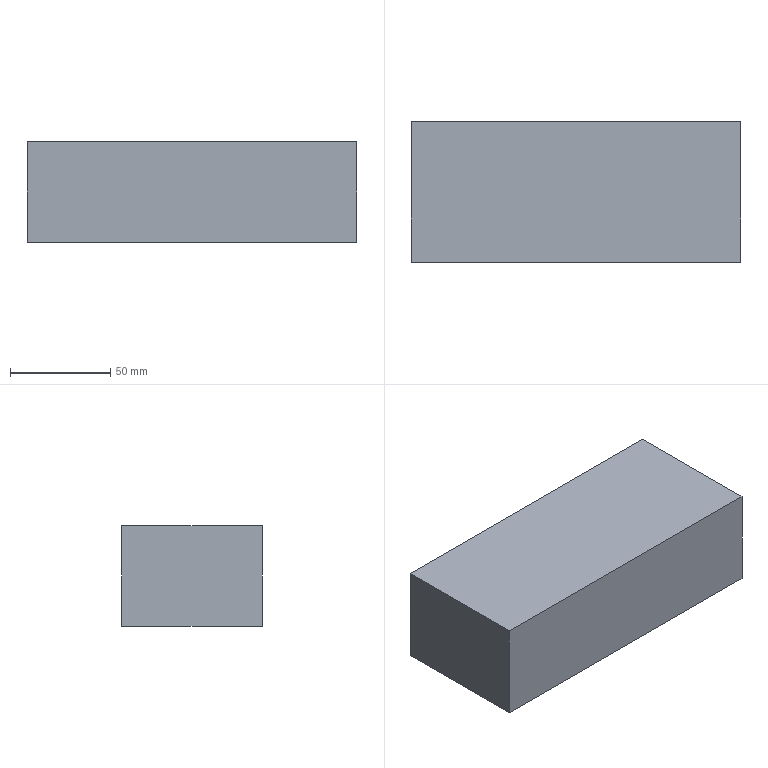Component | NX | PEN_HOLDER_BLOCK | 1 solid | 6 faces | box 164 x 70 x 50 mm | volume 574000 mm3 | plane 6
STEP:
#1=CARTESIAN_POINT('',(0.,0.,0.));
#2=DIRECTION('',(0.,0.,1.));
#3=DIRECTION('',(1.,0.,0.));
#4=AXIS2_PLACEMENT_3D('',#1,#2,#3);
#5=CARTESIAN_POINT('',(289.534,43.893,-32.704));
#6=VERTEX_POINT('',#5);
#7=CARTESIAN_POINT('',(289.534,43.893,17.296));
#8=VERTEX_POINT('',#7);
#9=CARTESIAN_POINT('',(289.534,43.893,-32.704));
#10=DIRECTION('',(0.,0.,1.));
#11=VECTOR('',#10,1.);
#12=LINE('',#9,#11);
#13=CARTESIAN_POINT('',(125.534,43.893,-32.704));
#14=DIRECTION('',(0.,1.,0.));
#15=DIRECTION('',(1.,0.,0.));
#16=AXIS2_PLACEMENT_3D('',#13,#14,#15);
#17=PLANE('',#16);
#18=CARTESIAN_POINT('',(164.,0.));
#19=DIRECTION('',(0.,-1.));
#20=VECTOR('',#19,1.);
#21=LINE('',#18,#20);
#22=(GEOMETRIC_REPRESENTATION_CONTEXT(2)PARAMETRIC_REPRESENTATION_CONTEXT()REPRESENTATION_CONTEXT('',''));
#23=DEFINITIONAL_REPRESENTATION('',(#21),#22);
#24=PCURVE('',#17,#23);
#25=CARTESIAN_POINT('',(289.534,103.893,-7.704));
#26=DIRECTION('',(-1.,0.,0.));
#27=DIRECTION('',(0.,1.,0.));
#28=AXIS2_PLACEMENT_3D('',#25,#26,#27);
#29=PLANE('',#28);
#30=CARTESIAN_POINT('',(-60.,25.));
#31=DIRECTION('',(0.,-1.));
#32=VECTOR('',#31,1.);
#33=LINE('',#30,#32);
#34=(GEOMETRIC_REPRESENTATION_CONTEXT(2)PARAMETRIC_REPRESENTATION_CONTEXT()REPRESENTATION_CONTEXT('',''));
#35=DEFINITIONAL_REPRESENTATION('',(#33),#34);
#36=PCURVE('',#29,#35);
#37=SURFACE_CURVE('',#12,(#24,#36),.PCURVE_S1.);
#38=EDGE_CURVE('',#6,#8,#37,.T.);
#39=ORIENTED_EDGE('',*,*,#38,.T.);
#40=CARTESIAN_POINT('',(125.534,43.893,17.296));
#41=VERTEX_POINT('',#40);
#42=CARTESIAN_POINT('',(125.534,43.893,17.296));
#43=DIRECTION('',(1.,0.,0.));
#44=VECTOR('',#43,1.);
#45=LINE('',#42,#44);
#46=CARTESIAN_POINT('',(0.,-50.));
#47=DIRECTION('',(1.,0.));
#48=VECTOR('',#47,1.);
#49=LINE('',#46,#48);
#50=(GEOMETRIC_REPRESENTATION_CONTEXT(2)PARAMETRIC_REPRESENTATION_CONTEXT()REPRESENTATION_CONTEXT('',''));
#51=DEFINITIONAL_REPRESENTATION('',(#49),#50);
#52=PCURVE('',#17,#51);
#53=CARTESIAN_POINT('',(125.534,43.893,17.296));
#54=DIRECTION('',(0.,0.,-1.));
#55=DIRECTION('',(-1.,0.,0.));
#56=AXIS2_PLACEMENT_3D('',#53,#54,#55);
#57=PLANE('',#56);
#58=CARTESIAN_POINT('',(0.,0.));
#59=DIRECTION('',(-1.,0.));
#60=VECTOR('',#59,1.);
#61=LINE('',#58,#60);
#62=(GEOMETRIC_REPRESENTATION_CONTEXT(2)PARAMETRIC_REPRESENTATION_CONTEXT()REPRESENTATION_CONTEXT('',''));
#63=DEFINITIONAL_REPRESENTATION('',(#61),#62);
#64=PCURVE('',#57,#63);
#65=SURFACE_CURVE('',#45,(#52,#64),.PCURVE_S1.);
#66=EDGE_CURVE('',#41,#8,#65,.T.);
#67=ORIENTED_EDGE('',*,*,#66,.F.);
#68=CARTESIAN_POINT('',(125.534,43.893,-32.704));
#69=VERTEX_POINT('',#68);
#70=CARTESIAN_POINT('',(125.534,43.893,-32.704));
#71=DIRECTION('',(0.,0.,1.));
#72=VECTOR('',#71,1.);
#73=LINE('',#70,#72);
#74=CARTESIAN_POINT('',(0.,0.));
#75=DIRECTION('',(0.,-1.));
#76=VECTOR('',#75,1.);
#77=LINE('',#74,#76);
#78=(GEOMETRIC_REPRESENTATION_CONTEXT(2)PARAMETRIC_REPRESENTATION_CONTEXT()REPRESENTATION_CONTEXT('',''));
#79=DEFINITIONAL_REPRESENTATION('',(#77),#78);
#80=PCURVE('',#17,#79);
#81=CARTESIAN_POINT('',(125.534,103.893,-7.704));
#82=DIRECTION('',(-1.,0.,0.));
#83=DIRECTION('',(0.,1.,0.));
#84=AXIS2_PLACEMENT_3D('',#81,#82,#83);
#85=PLANE('',#84);
#86=CARTESIAN_POINT('',(-60.,25.));
#87=DIRECTION('',(0.,-1.));
#88=VECTOR('',#87,1.);
#89=LINE('',#86,#88);
#90=(GEOMETRIC_REPRESENTATION_CONTEXT(2)PARAMETRIC_REPRESENTATION_CONTEXT()REPRESENTATION_CONTEXT('',''));
#91=DEFINITIONAL_REPRESENTATION('',(#89),#90);
#92=PCURVE('',#85,#91);
#93=SURFACE_CURVE('',#73,(#80,#92),.PCURVE_S1.);
#94=EDGE_CURVE('',#69,#41,#93,.T.);
#95=ORIENTED_EDGE('',*,*,#94,.F.);
#96=CARTESIAN_POINT('',(125.534,43.893,-32.704));
#97=DIRECTION('',(1.,0.,0.));
#98=VECTOR('',#97,1.);
#99=LINE('',#96,#98);
#100=CARTESIAN_POINT('',(0.,0.));
#101=DIRECTION('',(1.,0.));
#102=VECTOR('',#101,1.);
#103=LINE('',#100,#102);
#104=(GEOMETRIC_REPRESENTATION_CONTEXT(2)PARAMETRIC_REPRESENTATION_CONTEXT()REPRESENTATION_CONTEXT('',''));
#105=DEFINITIONAL_REPRESENTATION('',(#103),#104);
#106=PCURVE('',#17,#105);
#107=CARTESIAN_POINT('',(125.534,163.893,-32.704));
#108=DIRECTION('',(0.,0.,1.));
#109=DIRECTION('',(1.,0.,0.));
#110=AXIS2_PLACEMENT_3D('',#107,#108,#109);
#111=PLANE('',#110);
#112=CARTESIAN_POINT('',(0.,-120.));
#113=DIRECTION('',(1.,0.));
#114=VECTOR('',#113,1.);
#115=LINE('',#112,#114);
#116=(GEOMETRIC_REPRESENTATION_CONTEXT(2)PARAMETRIC_REPRESENTATION_CONTEXT()REPRESENTATION_CONTEXT('',''));
#117=DEFINITIONAL_REPRESENTATION('',(#115),#116);
#118=PCURVE('',#111,#117);
#119=SURFACE_CURVE('',#99,(#106,#118),.PCURVE_S1.);
#120=EDGE_CURVE('',#69,#6,#119,.T.);
#121=ORIENTED_EDGE('',*,*,#120,.T.);
#122=EDGE_LOOP('',(#39,#67,#95,#121));
#123=FACE_BOUND('',#122,.T.);
#124=ADVANCED_FACE('',(#123),#17,.F.);
#125=CARTESIAN_POINT('',(289.534,113.893,17.296));
#126=VERTEX_POINT('',#125);
#127=CARTESIAN_POINT('',(289.534,43.893,17.296));
#128=DIRECTION('',(0.,1.,0.));
#129=VECTOR('',#128,1.);
#130=LINE('',#127,#129);
#131=CARTESIAN_POINT('',(-164.,0.));
#132=DIRECTION('',(0.,1.));
#133=VECTOR('',#132,1.);
#134=LINE('',#131,#133);
#135=(GEOMETRIC_REPRESENTATION_CONTEXT(2)PARAMETRIC_REPRESENTATION_CONTEXT()REPRESENTATION_CONTEXT('',''));
#136=DEFINITIONAL_REPRESENTATION('',(#134),#135);
#137=PCURVE('',#57,#136);
#138=CARTESIAN_POINT('',(-60.,-25.));
#139=DIRECTION('',(1.,0.));
#140=VECTOR('',#139,1.);
#141=LINE('',#138,#140);
#142=(GEOMETRIC_REPRESENTATION_CONTEXT(2)PARAMETRIC_REPRESENTATION_CONTEXT()REPRESENTATION_CONTEXT('',''));
#143=DEFINITIONAL_REPRESENTATION('',(#141),#142);
#144=PCURVE('',#29,#143);
#145=SURFACE_CURVE('',#130,(#137,#144),.PCURVE_S1.);
#146=EDGE_CURVE('',#8,#126,#145,.T.);
#147=ORIENTED_EDGE('',*,*,#146,.T.);
#148=CARTESIAN_POINT('',(125.534,113.893,17.296));
#149=VERTEX_POINT('',#148);
#150=CARTESIAN_POINT('',(125.534,113.893,17.296));
#151=DIRECTION('',(1.,0.,0.));
#152=VECTOR('',#151,1.);
#153=LINE('',#150,#152);
#154=CARTESIAN_POINT('',(0.,70.));
#155=DIRECTION('',(-1.,0.));
#156=VECTOR('',#155,1.);
#157=LINE('',#154,#156);
#158=(GEOMETRIC_REPRESENTATION_CONTEXT(2)PARAMETRIC_REPRESENTATION_CONTEXT()REPRESENTATION_CONTEXT('',''));
#159=DEFINITIONAL_REPRESENTATION('',(#157),#158);
#160=PCURVE('',#57,#159);
#161=CARTESIAN_POINT('',(125.534,113.893,17.296));
#162=DIRECTION('',(0.,-1.,0.));
#163=DIRECTION('',(-1.,0.,0.));
#164=AXIS2_PLACEMENT_3D('',#161,#162,#163);
#165=PLANE('',#164);
#166=CARTESIAN_POINT('',(0.,0.));
#167=DIRECTION('',(-1.,0.));
#168=VECTOR('',#167,1.);
#169=LINE('',#166,#168);
#170=(GEOMETRIC_REPRESENTATION_CONTEXT(2)PARAMETRIC_REPRESENTATION_CONTEXT()REPRESENTATION_CONTEXT('',''));
#171=DEFINITIONAL_REPRESENTATION('',(#169),#170);
#172=PCURVE('',#165,#171);
#173=SURFACE_CURVE('',#153,(#160,#172),.PCURVE_S1.);
#174=EDGE_CURVE('',#149,#126,#173,.T.);
#175=ORIENTED_EDGE('',*,*,#174,.F.);
#176=CARTESIAN_POINT('',(125.534,43.893,17.296));
#177=DIRECTION('',(0.,1.,0.));
#178=VECTOR('',#177,1.);
#179=LINE('',#176,#178);
#180=CARTESIAN_POINT('',(0.,0.));
#181=DIRECTION('',(0.,1.));
#182=VECTOR('',#181,1.);
#183=LINE('',#180,#182);
#184=(GEOMETRIC_REPRESENTATION_CONTEXT(2)PARAMETRIC_REPRESENTATION_CONTEXT()REPRESENTATION_CONTEXT('',''));
#185=DEFINITIONAL_REPRESENTATION('',(#183),#184);
#186=PCURVE('',#57,#185);
#187=CARTESIAN_POINT('',(-60.,-25.));
#188=DIRECTION('',(1.,0.));
#189=VECTOR('',#188,1.);
#190=LINE('',#187,#189);
#191=(GEOMETRIC_REPRESENTATION_CONTEXT(2)PARAMETRIC_REPRESENTATION_CONTEXT()REPRESENTATION_CONTEXT('',''));
#192=DEFINITIONAL_REPRESENTATION('',(#190),#191);
#193=PCURVE('',#85,#192);
#194=SURFACE_CURVE('',#179,(#186,#193),.PCURVE_S1.);
#195=EDGE_CURVE('',#41,#149,#194,.T.);
#196=ORIENTED_EDGE('',*,*,#195,.F.);
#197=ORIENTED_EDGE('',*,*,#66,.T.);
#198=EDGE_LOOP('',(#147,#175,#196,#197));
#199=FACE_BOUND('',#198,.T.);
#200=ADVANCED_FACE('',(#199),#57,.F.);
#201=CARTESIAN_POINT('',(289.534,113.893,-32.704));
#202=VERTEX_POINT('',#201);
#203=CARTESIAN_POINT('',(289.534,113.893,17.296));
#204=DIRECTION('',(0.,0.,-1.));
#205=VECTOR('',#204,1.);
#206=LINE('',#203,#205);
#207=CARTESIAN_POINT('',(-164.,0.));
#208=DIRECTION('',(0.,1.));
#209=VECTOR('',#208,1.);
#210=LINE('',#207,#209);
#211=(GEOMETRIC_REPRESENTATION_CONTEXT(2)PARAMETRIC_REPRESENTATION_CONTEXT()REPRESENTATION_CONTEXT('',''));
#212=DEFINITIONAL_REPRESENTATION('',(#210),#211);
#213=PCURVE('',#165,#212);
#214=CARTESIAN_POINT('',(10.,-25.));
#215=DIRECTION('',(0.,1.));
#216=VECTOR('',#215,1.);
#217=LINE('',#214,#216);
#218=(GEOMETRIC_REPRESENTATION_CONTEXT(2)PARAMETRIC_REPRESENTATION_CONTEXT()REPRESENTATION_CONTEXT('',''));
#219=DEFINITIONAL_REPRESENTATION('',(#217),#218);
#220=PCURVE('',#29,#219);
#221=SURFACE_CURVE('',#206,(#213,#220),.PCURVE_S1.);
#222=EDGE_CURVE('',#126,#202,#221,.T.);
#223=ORIENTED_EDGE('',*,*,#222,.T.);
#224=CARTESIAN_POINT('',(125.534,113.893,-32.704));
#225=VERTEX_POINT('',#224);
#226=CARTESIAN_POINT('',(125.534,113.893,-32.704));
#227=DIRECTION('',(1.,0.,0.));
#228=VECTOR('',#227,1.);
#229=LINE('',#226,#228);
#230=CARTESIAN_POINT('',(0.,50.));
#231=DIRECTION('',(-1.,0.));
#232=VECTOR('',#231,1.);
#233=LINE('',#230,#232);
#234=(GEOMETRIC_REPRESENTATION_CONTEXT(2)PARAMETRIC_REPRESENTATION_CONTEXT()REPRESENTATION_CONTEXT('',''));
#235=DEFINITIONAL_REPRESENTATION('',(#233),#234);
#236=PCURVE('',#165,#235);
#237=CARTESIAN_POINT('',(0.,-50.));
#238=DIRECTION('',(1.,0.));
#239=VECTOR('',#238,1.);
#240=LINE('',#237,#239);
#241=(GEOMETRIC_REPRESENTATION_CONTEXT(2)PARAMETRIC_REPRESENTATION_CONTEXT()REPRESENTATION_CONTEXT('',''));
#242=DEFINITIONAL_REPRESENTATION('',(#240),#241);
#243=PCURVE('',#111,#242);
#244=SURFACE_CURVE('',#229,(#236,#243),.PCURVE_S1.);
#245=EDGE_CURVE('',#225,#202,#244,.T.);
#246=ORIENTED_EDGE('',*,*,#245,.F.);
#247=CARTESIAN_POINT('',(125.534,113.893,17.296));
#248=DIRECTION('',(0.,0.,-1.));
#249=VECTOR('',#248,1.);
#250=LINE('',#247,#249);
#251=CARTESIAN_POINT('',(0.,0.));
#252=DIRECTION('',(0.,1.));
#253=VECTOR('',#252,1.);
#254=LINE('',#251,#253);
#255=(GEOMETRIC_REPRESENTATION_CONTEXT(2)PARAMETRIC_REPRESENTATION_CONTEXT()REPRESENTATION_CONTEXT('',''));
#256=DEFINITIONAL_REPRESENTATION('',(#254),#255);
#257=PCURVE('',#165,#256);
#258=CARTESIAN_POINT('',(10.,-25.));
#259=DIRECTION('',(0.,1.));
#260=VECTOR('',#259,1.);
#261=LINE('',#258,#260);
#262=(GEOMETRIC_REPRESENTATION_CONTEXT(2)PARAMETRIC_REPRESENTATION_CONTEXT()REPRESENTATION_CONTEXT('',''));
#263=DEFINITIONAL_REPRESENTATION('',(#261),#262);
#264=PCURVE('',#85,#263);
#265=SURFACE_CURVE('',#250,(#257,#264),.PCURVE_S1.);
#266=EDGE_CURVE('',#149,#225,#265,.T.);
#267=ORIENTED_EDGE('',*,*,#266,.F.);
#268=ORIENTED_EDGE('',*,*,#174,.T.);
#269=EDGE_LOOP('',(#223,#246,#267,#268));
#270=FACE_BOUND('',#269,.T.);
#271=ADVANCED_FACE('',(#270),#165,.F.);
#272=CARTESIAN_POINT('',(289.534,163.893,-32.704));
#273=DIRECTION('',(0.,-1.,0.));
#274=VECTOR('',#273,1.);
#275=LINE('',#272,#274);
#276=CARTESIAN_POINT('',(164.,0.));
#277=DIRECTION('',(0.,-1.));
#278=VECTOR('',#277,1.);
#279=LINE('',#276,#278);
#280=(GEOMETRIC_REPRESENTATION_CONTEXT(2)PARAMETRIC_REPRESENTATION_CONTEXT()REPRESENTATION_CONTEXT('',''));
#281=DEFINITIONAL_REPRESENTATION('',(#279),#280);
#282=PCURVE('',#111,#281);
#283=CARTESIAN_POINT('',(60.,25.));
#284=DIRECTION('',(-1.,0.));
#285=VECTOR('',#284,1.);
#286=LINE('',#283,#285);
#287=(GEOMETRIC_REPRESENTATION_CONTEXT(2)PARAMETRIC_REPRESENTATION_CONTEXT()REPRESENTATION_CONTEXT('',''));
#288=DEFINITIONAL_REPRESENTATION('',(#286),#287);
#289=PCURVE('',#29,#288);
#290=SURFACE_CURVE('',#275,(#282,#289),.PCURVE_S1.);
#291=EDGE_CURVE('',#202,#6,#290,.T.);
#292=ORIENTED_EDGE('',*,*,#291,.T.);
#293=ORIENTED_EDGE('',*,*,#120,.F.);
#294=CARTESIAN_POINT('',(125.534,163.893,-32.704));
#295=DIRECTION('',(0.,-1.,0.));
#296=VECTOR('',#295,1.);
#297=LINE('',#294,#296);
#298=CARTESIAN_POINT('',(0.,0.));
#299=DIRECTION('',(0.,-1.));
#300=VECTOR('',#299,1.);
#301=LINE('',#298,#300);
#302=(GEOMETRIC_REPRESENTATION_CONTEXT(2)PARAMETRIC_REPRESENTATION_CONTEXT()REPRESENTATION_CONTEXT('',''));
#303=DEFINITIONAL_REPRESENTATION('',(#301),#302);
#304=PCURVE('',#111,#303);
#305=CARTESIAN_POINT('',(60.,25.));
#306=DIRECTION('',(-1.,0.));
#307=VECTOR('',#306,1.);
#308=LINE('',#305,#307);
#309=(GEOMETRIC_REPRESENTATION_CONTEXT(2)PARAMETRIC_REPRESENTATION_CONTEXT()REPRESENTATION_CONTEXT('',''));
#310=DEFINITIONAL_REPRESENTATION('',(#308),#309);
#311=PCURVE('',#85,#310);
#312=SURFACE_CURVE('',#297,(#304,#311),.PCURVE_S1.);
#313=EDGE_CURVE('',#225,#69,#312,.T.);
#314=ORIENTED_EDGE('',*,*,#313,.F.);
#315=ORIENTED_EDGE('',*,*,#245,.T.);
#316=EDGE_LOOP('',(#292,#293,#314,#315));
#317=FACE_BOUND('',#316,.T.);
#318=ADVANCED_FACE('',(#317),#111,.F.);
#319=ORIENTED_EDGE('',*,*,#94,.T.);
#320=ORIENTED_EDGE('',*,*,#195,.T.);
#321=ORIENTED_EDGE('',*,*,#266,.T.);
#322=ORIENTED_EDGE('',*,*,#313,.T.);
#323=EDGE_LOOP('',(#319,#320,#321,#322));
#324=FACE_BOUND('',#323,.T.);
#325=ADVANCED_FACE('',(#324),#85,.T.);
#326=ORIENTED_EDGE('',*,*,#38,.F.);
#327=ORIENTED_EDGE('',*,*,#291,.F.);
#328=ORIENTED_EDGE('',*,*,#222,.F.);
#329=ORIENTED_EDGE('',*,*,#146,.F.);
#330=EDGE_LOOP('',(#326,#327,#328,#329));
#331=FACE_BOUND('',#330,.T.);
#332=ADVANCED_FACE('',(#331),#29,.F.);
#333=CLOSED_SHELL('',(#124,#200,#271,#318,#325,#332));
#334=MANIFOLD_SOLID_BREP('',#333);
#335=(LENGTH_UNIT()NAMED_UNIT(*)SI_UNIT(.MILLI.,.METRE.));
#336=UNCERTAINTY_MEASURE_WITH_UNIT(LENGTH_MEASURE(0.0000001),#335,'','');
#337=(NAMED_UNIT(*)PLANE_ANGLE_UNIT()SI_UNIT($,.RADIAN.));
#338=(NAMED_UNIT(*)SI_UNIT($,.STERADIAN.)SOLID_ANGLE_UNIT());
#339=(GEOMETRIC_REPRESENTATION_CONTEXT(3)GLOBAL_UNCERTAINTY_ASSIGNED_CONTEXT((#336))GLOBAL_UNIT_ASSIGNED_CONTEXT((#335,#337,#338))REPRESENTATION_CONTEXT('',''));
#340=ADVANCED_BREP_SHAPE_REPRESENTATION('',(#4,#334),#339);